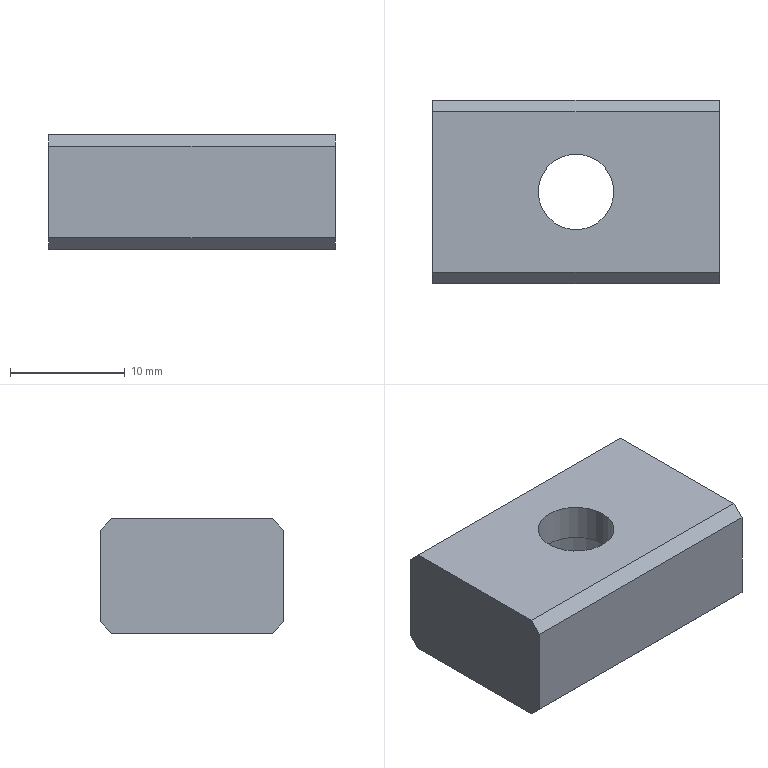Component | NX | LOCATING_KEY | 1 solid | 13 faces | box 25 x 16 x 10 mm | volume 3194 mm3 | plane 11 | cylinder 2 | commonest cylinder face diameters 6.6 x1 11 x1
STEP:
#1=CARTESIAN_POINT('',(0.,0.,0.));
#2=DIRECTION('',(0.,0.,1.));
#3=DIRECTION('',(1.,0.,0.));
#4=AXIS2_PLACEMENT_3D('',#1,#2,#3);
#5=CARTESIAN_POINT('',(225.,7.,-35.));
#6=VERTEX_POINT('',#5);
#7=CARTESIAN_POINT('',(225.,-7.,-35.));
#8=VERTEX_POINT('',#7);
#9=CARTESIAN_POINT('',(225.,8.,-35.));
#10=DIRECTION('',(0.,-1.,0.));
#11=VECTOR('',#10,1.);
#12=LINE('',#9,#11);
#13=CARTESIAN_POINT('',(225.,8.,-35.));
#14=DIRECTION('',(1.,0.,0.));
#15=DIRECTION('',(0.,0.,-1.));
#16=AXIS2_PLACEMENT_3D('',#13,#14,#15);
#17=PLANE('',#16);
#18=CARTESIAN_POINT('',(0.,0.));
#19=DIRECTION('',(0.,-1.));
#20=VECTOR('',#19,1.);
#21=LINE('',#18,#20);
#22=(GEOMETRIC_REPRESENTATION_CONTEXT(2)PARAMETRIC_REPRESENTATION_CONTEXT()REPRESENTATION_CONTEXT('',''));
#23=DEFINITIONAL_REPRESENTATION('',(#21),#22);
#24=PCURVE('',#17,#23);
#25=CARTESIAN_POINT('',(237.5,-0.,-35.));
#26=DIRECTION('',(0.,0.,1.));
#27=DIRECTION('',(1.,0.,0.));
#28=AXIS2_PLACEMENT_3D('',#25,#26,#27);
#29=PLANE('',#28);
#30=CARTESIAN_POINT('',(-12.5,8.));
#31=DIRECTION('',(0.,-1.));
#32=VECTOR('',#31,1.);
#33=LINE('',#30,#32);
#34=(GEOMETRIC_REPRESENTATION_CONTEXT(2)PARAMETRIC_REPRESENTATION_CONTEXT()REPRESENTATION_CONTEXT('',''));
#35=DEFINITIONAL_REPRESENTATION('',(#33),#34);
#36=PCURVE('',#29,#35);
#37=SURFACE_CURVE('',#12,(#24,#36),.PCURVE_S1.);
#38=EDGE_CURVE('',#6,#8,#37,.T.);
#39=ORIENTED_EDGE('',*,*,#38,.F.);
#40=CARTESIAN_POINT('',(225.,8.,-36.));
#41=VERTEX_POINT('',#40);
#42=CARTESIAN_POINT('',(225.,7.,-35.));
#43=DIRECTION('',(0.,0.7071,-0.7071));
#44=VECTOR('',#43,1.);
#45=LINE('',#42,#44);
#46=CARTESIAN_POINT('',(0.,-1.));
#47=DIRECTION('',(0.7071,0.7071));
#48=VECTOR('',#47,1.);
#49=LINE('',#46,#48);
#50=(GEOMETRIC_REPRESENTATION_CONTEXT(2)PARAMETRIC_REPRESENTATION_CONTEXT()REPRESENTATION_CONTEXT('',''));
#51=DEFINITIONAL_REPRESENTATION('',(#49),#50);
#52=PCURVE('',#17,#51);
#53=CARTESIAN_POINT('',(237.5,7.,-35.));
#54=DIRECTION('',(0.,0.7071,0.7071));
#55=DIRECTION('',(1.,0.,0.));
#56=AXIS2_PLACEMENT_3D('',#53,#54,#55);
#57=PLANE('',#56);
#58=CARTESIAN_POINT('',(-12.5,0.));
#59=DIRECTION('',(0.,1.));
#60=VECTOR('',#59,1.);
#61=LINE('',#58,#60);
#62=(GEOMETRIC_REPRESENTATION_CONTEXT(2)PARAMETRIC_REPRESENTATION_CONTEXT()REPRESENTATION_CONTEXT('',''));
#63=DEFINITIONAL_REPRESENTATION('',(#61),#62);
#64=PCURVE('',#57,#63);
#65=SURFACE_CURVE('',#45,(#52,#64),.PCURVE_S1.);
#66=EDGE_CURVE('',#6,#41,#65,.T.);
#67=ORIENTED_EDGE('',*,*,#66,.T.);
#68=CARTESIAN_POINT('',(225.,8.,-44.));
#69=VERTEX_POINT('',#68);
#70=CARTESIAN_POINT('',(225.,8.,-35.));
#71=DIRECTION('',(0.,0.,-1.));
#72=VECTOR('',#71,1.);
#73=LINE('',#70,#72);
#74=CARTESIAN_POINT('',(0.,0.));
#75=DIRECTION('',(1.,0.));
#76=VECTOR('',#75,1.);
#77=LINE('',#74,#76);
#78=(GEOMETRIC_REPRESENTATION_CONTEXT(2)PARAMETRIC_REPRESENTATION_CONTEXT()REPRESENTATION_CONTEXT('',''));
#79=DEFINITIONAL_REPRESENTATION('',(#77),#78);
#80=PCURVE('',#17,#79);
#81=CARTESIAN_POINT('',(250.,8.,-35.));
#82=DIRECTION('',(0.,-1.,0.));
#83=DIRECTION('',(0.,0.,-1.));
#84=AXIS2_PLACEMENT_3D('',#81,#82,#83);
#85=PLANE('',#84);
#86=CARTESIAN_POINT('',(0.,-25.));
#87=DIRECTION('',(1.,0.));
#88=VECTOR('',#87,1.);
#89=LINE('',#86,#88);
#90=(GEOMETRIC_REPRESENTATION_CONTEXT(2)PARAMETRIC_REPRESENTATION_CONTEXT()REPRESENTATION_CONTEXT('',''));
#91=DEFINITIONAL_REPRESENTATION('',(#89),#90);
#92=PCURVE('',#85,#91);
#93=SURFACE_CURVE('',#73,(#80,#92),.PCURVE_S1.);
#94=EDGE_CURVE('',#41,#69,#93,.T.);
#95=ORIENTED_EDGE('',*,*,#94,.T.);
#96=CARTESIAN_POINT('',(225.,7.,-45.));
#97=VERTEX_POINT('',#96);
#98=CARTESIAN_POINT('',(225.,8.,-44.));
#99=DIRECTION('',(0.,-0.7071,-0.7071));
#100=VECTOR('',#99,1.);
#101=LINE('',#98,#100);
#102=CARTESIAN_POINT('',(9.,0.));
#103=DIRECTION('',(0.7071,-0.7071));
#104=VECTOR('',#103,1.);
#105=LINE('',#102,#104);
#106=(GEOMETRIC_REPRESENTATION_CONTEXT(2)PARAMETRIC_REPRESENTATION_CONTEXT()REPRESENTATION_CONTEXT('',''));
#107=DEFINITIONAL_REPRESENTATION('',(#105),#106);
#108=PCURVE('',#17,#107);
#109=CARTESIAN_POINT('',(250.,8.,-44.));
#110=DIRECTION('',(0.,-0.7071,0.7071));
#111=DIRECTION('',(-1.,0.,0.));
#112=AXIS2_PLACEMENT_3D('',#109,#110,#111);
#113=PLANE('',#112);
#114=CARTESIAN_POINT('',(25.,0.));
#115=DIRECTION('',(0.,1.));
#116=VECTOR('',#115,1.);
#117=LINE('',#114,#116);
#118=(GEOMETRIC_REPRESENTATION_CONTEXT(2)PARAMETRIC_REPRESENTATION_CONTEXT()REPRESENTATION_CONTEXT('',''));
#119=DEFINITIONAL_REPRESENTATION('',(#117),#118);
#120=PCURVE('',#113,#119);
#121=SURFACE_CURVE('',#101,(#108,#120),.PCURVE_S1.);
#122=EDGE_CURVE('',#69,#97,#121,.T.);
#123=ORIENTED_EDGE('',*,*,#122,.T.);
#124=CARTESIAN_POINT('',(225.,-7.,-45.));
#125=VERTEX_POINT('',#124);
#126=CARTESIAN_POINT('',(225.,8.,-45.));
#127=DIRECTION('',(0.,-1.,0.));
#128=VECTOR('',#127,1.);
#129=LINE('',#126,#128);
#130=CARTESIAN_POINT('',(10.,0.));
#131=DIRECTION('',(0.,-1.));
#132=VECTOR('',#131,1.);
#133=LINE('',#130,#132);
#134=(GEOMETRIC_REPRESENTATION_CONTEXT(2)PARAMETRIC_REPRESENTATION_CONTEXT()REPRESENTATION_CONTEXT('',''));
#135=DEFINITIONAL_REPRESENTATION('',(#133),#134);
#136=PCURVE('',#17,#135);
#137=CARTESIAN_POINT('',(237.5,-0.,-45.));
#138=DIRECTION('',(0.,0.,1.));
#139=DIRECTION('',(1.,0.,0.));
#140=AXIS2_PLACEMENT_3D('',#137,#138,#139);
#141=PLANE('',#140);
#142=CARTESIAN_POINT('',(-12.5,8.));
#143=DIRECTION('',(0.,-1.));
#144=VECTOR('',#143,1.);
#145=LINE('',#142,#144);
#146=(GEOMETRIC_REPRESENTATION_CONTEXT(2)PARAMETRIC_REPRESENTATION_CONTEXT()REPRESENTATION_CONTEXT('',''));
#147=DEFINITIONAL_REPRESENTATION('',(#145),#146);
#148=PCURVE('',#141,#147);
#149=SURFACE_CURVE('',#129,(#136,#148),.PCURVE_S1.);
#150=EDGE_CURVE('',#97,#125,#149,.T.);
#151=ORIENTED_EDGE('',*,*,#150,.T.);
#152=CARTESIAN_POINT('',(225.,-8.,-44.));
#153=VERTEX_POINT('',#152);
#154=CARTESIAN_POINT('',(225.,-8.,-44.));
#155=DIRECTION('',(0.,-0.7071,0.7071));
#156=VECTOR('',#155,1.);
#157=LINE('',#154,#156);
#158=CARTESIAN_POINT('',(9.,-16.));
#159=DIRECTION('',(-0.7071,-0.7071));
#160=VECTOR('',#159,1.);
#161=LINE('',#158,#160);
#162=(GEOMETRIC_REPRESENTATION_CONTEXT(2)PARAMETRIC_REPRESENTATION_CONTEXT()REPRESENTATION_CONTEXT('',''));
#163=DEFINITIONAL_REPRESENTATION('',(#161),#162);
#164=PCURVE('',#17,#163);
#165=CARTESIAN_POINT('',(225.,-8.,-44.));
#166=DIRECTION('',(0.,0.7071,0.7071));
#167=DIRECTION('',(1.,0.,0.));
#168=AXIS2_PLACEMENT_3D('',#165,#166,#167);
#169=PLANE('',#168);
#170=CARTESIAN_POINT('',(0.,0.));
#171=DIRECTION('',(0.,-1.));
#172=VECTOR('',#171,1.);
#173=LINE('',#170,#172);
#174=(GEOMETRIC_REPRESENTATION_CONTEXT(2)PARAMETRIC_REPRESENTATION_CONTEXT()REPRESENTATION_CONTEXT('',''));
#175=DEFINITIONAL_REPRESENTATION('',(#173),#174);
#176=PCURVE('',#169,#175);
#177=SURFACE_CURVE('',#157,(#164,#176),.PCURVE_S1.);
#178=EDGE_CURVE('',#125,#153,#177,.T.);
#179=ORIENTED_EDGE('',*,*,#178,.T.);
#180=CARTESIAN_POINT('',(225.,-8.,-36.));
#181=VERTEX_POINT('',#180);
#182=CARTESIAN_POINT('',(225.,-8.,-35.));
#183=DIRECTION('',(0.,0.,-1.));
#184=VECTOR('',#183,1.);
#185=LINE('',#182,#184);
#186=CARTESIAN_POINT('',(0.,-16.));
#187=DIRECTION('',(1.,0.));
#188=VECTOR('',#187,1.);
#189=LINE('',#186,#188);
#190=(GEOMETRIC_REPRESENTATION_CONTEXT(2)PARAMETRIC_REPRESENTATION_CONTEXT()REPRESENTATION_CONTEXT('',''));
#191=DEFINITIONAL_REPRESENTATION('',(#189),#190);
#192=PCURVE('',#17,#191);
#193=CARTESIAN_POINT('',(225.,-8.,-35.));
#194=DIRECTION('',(0.,1.,0.));
#195=DIRECTION('',(0.,0.,1.));
#196=AXIS2_PLACEMENT_3D('',#193,#194,#195);
#197=PLANE('',#196);
#198=CARTESIAN_POINT('',(0.,0.));
#199=DIRECTION('',(-1.,0.));
#200=VECTOR('',#199,1.);
#201=LINE('',#198,#200);
#202=(GEOMETRIC_REPRESENTATION_CONTEXT(2)PARAMETRIC_REPRESENTATION_CONTEXT()REPRESENTATION_CONTEXT('',''));
#203=DEFINITIONAL_REPRESENTATION('',(#201),#202);
#204=PCURVE('',#197,#203);
#205=SURFACE_CURVE('',#185,(#192,#204),.PCURVE_S1.);
#206=EDGE_CURVE('',#181,#153,#205,.T.);
#207=ORIENTED_EDGE('',*,*,#206,.F.);
#208=CARTESIAN_POINT('',(225.,-7.,-35.));
#209=DIRECTION('',(0.,0.7071,0.7071));
#210=VECTOR('',#209,1.);
#211=LINE('',#208,#210);
#212=CARTESIAN_POINT('',(0.,-15.));
#213=DIRECTION('',(-0.7071,0.7071));
#214=VECTOR('',#213,1.);
#215=LINE('',#212,#214);
#216=(GEOMETRIC_REPRESENTATION_CONTEXT(2)PARAMETRIC_REPRESENTATION_CONTEXT()REPRESENTATION_CONTEXT('',''));
#217=DEFINITIONAL_REPRESENTATION('',(#215),#216);
#218=PCURVE('',#17,#217);
#219=CARTESIAN_POINT('',(237.5,-7.,-35.));
#220=DIRECTION('',(0.,-0.7071,0.7071));
#221=DIRECTION('',(-1.,0.,0.));
#222=AXIS2_PLACEMENT_3D('',#219,#220,#221);
#223=PLANE('',#222);
#224=CARTESIAN_POINT('',(12.5,0.));
#225=DIRECTION('',(0.,-1.));
#226=VECTOR('',#225,1.);
#227=LINE('',#224,#226);
#228=(GEOMETRIC_REPRESENTATION_CONTEXT(2)PARAMETRIC_REPRESENTATION_CONTEXT()REPRESENTATION_CONTEXT('',''));
#229=DEFINITIONAL_REPRESENTATION('',(#227),#228);
#230=PCURVE('',#223,#229);
#231=SURFACE_CURVE('',#211,(#218,#230),.PCURVE_S1.);
#232=EDGE_CURVE('',#181,#8,#231,.T.);
#233=ORIENTED_EDGE('',*,*,#232,.T.);
#234=EDGE_LOOP('',(#39,#67,#95,#123,#151,#179,#207,#233));
#235=FACE_BOUND('',#234,.T.);
#236=ADVANCED_FACE('',(#235),#17,.F.);
#237=ORIENTED_EDGE('',*,*,#206,.T.);
#238=CARTESIAN_POINT('',(250.,-8.,-44.));
#239=VERTEX_POINT('',#238);
#240=CARTESIAN_POINT('',(225.,-8.,-44.));
#241=DIRECTION('',(1.,0.,0.));
#242=VECTOR('',#241,1.);
#243=LINE('',#240,#242);
#244=CARTESIAN_POINT('',(-9.,0.));
#245=DIRECTION('',(0.,1.));
#246=VECTOR('',#245,1.);
#247=LINE('',#244,#246);
#248=(GEOMETRIC_REPRESENTATION_CONTEXT(2)PARAMETRIC_REPRESENTATION_CONTEXT()REPRESENTATION_CONTEXT('',''));
#249=DEFINITIONAL_REPRESENTATION('',(#247),#248);
#250=PCURVE('',#197,#249);
#251=CARTESIAN_POINT('',(0.,0.));
#252=DIRECTION('',(1.,0.));
#253=VECTOR('',#252,1.);
#254=LINE('',#251,#253);
#255=(GEOMETRIC_REPRESENTATION_CONTEXT(2)PARAMETRIC_REPRESENTATION_CONTEXT()REPRESENTATION_CONTEXT('',''));
#256=DEFINITIONAL_REPRESENTATION('',(#254),#255);
#257=PCURVE('',#169,#256);
#258=SURFACE_CURVE('',#243,(#250,#257),.PCURVE_S1.);
#259=EDGE_CURVE('',#153,#239,#258,.T.);
#260=ORIENTED_EDGE('',*,*,#259,.T.);
#261=CARTESIAN_POINT('',(250.,-8.,-36.));
#262=VERTEX_POINT('',#261);
#263=CARTESIAN_POINT('',(250.,-8.,-35.));
#264=DIRECTION('',(0.,0.,-1.));
#265=VECTOR('',#264,1.);
#266=LINE('',#263,#265);
#267=CARTESIAN_POINT('',(0.,25.));
#268=DIRECTION('',(-1.,0.));
#269=VECTOR('',#268,1.);
#270=LINE('',#267,#269);
#271=(GEOMETRIC_REPRESENTATION_CONTEXT(2)PARAMETRIC_REPRESENTATION_CONTEXT()REPRESENTATION_CONTEXT('',''));
#272=DEFINITIONAL_REPRESENTATION('',(#270),#271);
#273=PCURVE('',#197,#272);
#274=CARTESIAN_POINT('',(250.,-8.,-35.));
#275=DIRECTION('',(-1.,0.,0.));
#276=DIRECTION('',(0.,0.,1.));
#277=AXIS2_PLACEMENT_3D('',#274,#275,#276);
#278=PLANE('',#277);
#279=CARTESIAN_POINT('',(0.,0.));
#280=DIRECTION('',(-1.,0.));
#281=VECTOR('',#280,1.);
#282=LINE('',#279,#281);
#283=(GEOMETRIC_REPRESENTATION_CONTEXT(2)PARAMETRIC_REPRESENTATION_CONTEXT()REPRESENTATION_CONTEXT('',''));
#284=DEFINITIONAL_REPRESENTATION('',(#282),#283);
#285=PCURVE('',#278,#284);
#286=SURFACE_CURVE('',#266,(#273,#285),.PCURVE_S1.);
#287=EDGE_CURVE('',#262,#239,#286,.T.);
#288=ORIENTED_EDGE('',*,*,#287,.F.);
#289=CARTESIAN_POINT('',(225.,-8.,-36.));
#290=DIRECTION('',(-1.,0.,0.));
#291=VECTOR('',#290,1.);
#292=LINE('',#289,#291);
#293=CARTESIAN_POINT('',(-1.,0.));
#294=DIRECTION('',(0.,-1.));
#295=VECTOR('',#294,1.);
#296=LINE('',#293,#295);
#297=(GEOMETRIC_REPRESENTATION_CONTEXT(2)PARAMETRIC_REPRESENTATION_CONTEXT()REPRESENTATION_CONTEXT('',''));
#298=DEFINITIONAL_REPRESENTATION('',(#296),#297);
#299=PCURVE('',#197,#298);
#300=CARTESIAN_POINT('',(12.5,1.414));
#301=DIRECTION('',(1.,0.));
#302=VECTOR('',#301,1.);
#303=LINE('',#300,#302);
#304=(GEOMETRIC_REPRESENTATION_CONTEXT(2)PARAMETRIC_REPRESENTATION_CONTEXT()REPRESENTATION_CONTEXT('',''));
#305=DEFINITIONAL_REPRESENTATION('',(#303),#304);
#306=PCURVE('',#223,#305);
#307=SURFACE_CURVE('',#292,(#299,#306),.PCURVE_S1.);
#308=EDGE_CURVE('',#262,#181,#307,.T.);
#309=ORIENTED_EDGE('',*,*,#308,.T.);
#310=EDGE_LOOP('',(#237,#260,#288,#309));
#311=FACE_BOUND('',#310,.T.);
#312=ADVANCED_FACE('',(#311),#197,.F.);
#313=CARTESIAN_POINT('',(250.,8.,-36.));
#314=VERTEX_POINT('',#313);
#315=CARTESIAN_POINT('',(250.,8.,-44.));
#316=VERTEX_POINT('',#315);
#317=CARTESIAN_POINT('',(250.,8.,-35.));
#318=DIRECTION('',(0.,0.,-1.));
#319=VECTOR('',#318,1.);
#320=LINE('',#317,#319);
#321=CARTESIAN_POINT('',(0.,16.));
#322=DIRECTION('',(-1.,0.));
#323=VECTOR('',#322,1.);
#324=LINE('',#321,#323);
#325=(GEOMETRIC_REPRESENTATION_CONTEXT(2)PARAMETRIC_REPRESENTATION_CONTEXT()REPRESENTATION_CONTEXT('',''));
#326=DEFINITIONAL_REPRESENTATION('',(#324),#325);
#327=PCURVE('',#278,#326);
#328=CARTESIAN_POINT('',(0.,0.));
#329=DIRECTION('',(1.,0.));
#330=VECTOR('',#329,1.);
#331=LINE('',#328,#330);
#332=(GEOMETRIC_REPRESENTATION_CONTEXT(2)PARAMETRIC_REPRESENTATION_CONTEXT()REPRESENTATION_CONTEXT('',''));
#333=DEFINITIONAL_REPRESENTATION('',(#331),#332);
#334=PCURVE('',#85,#333);
#335=SURFACE_CURVE('',#320,(#327,#334),.PCURVE_S1.);
#336=EDGE_CURVE('',#314,#316,#335,.T.);
#337=ORIENTED_EDGE('',*,*,#336,.F.);
#338=CARTESIAN_POINT('',(250.,7.,-35.));
#339=VERTEX_POINT('',#338);
#340=CARTESIAN_POINT('',(250.,7.,-35.));
#341=DIRECTION('',(0.,-0.7071,0.7071));
#342=VECTOR('',#341,1.);
#343=LINE('',#340,#342);
#344=CARTESIAN_POINT('',(0.,15.));
#345=DIRECTION('',(0.7071,-0.7071));
#346=VECTOR('',#345,1.);
#347=LINE('',#344,#346);
#348=(GEOMETRIC_REPRESENTATION_CONTEXT(2)PARAMETRIC_REPRESENTATION_CONTEXT()REPRESENTATION_CONTEXT('',''));
#349=DEFINITIONAL_REPRESENTATION('',(#347),#348);
#350=PCURVE('',#278,#349);
#351=CARTESIAN_POINT('',(12.5,0.));
#352=DIRECTION('',(0.,-1.));
#353=VECTOR('',#352,1.);
#354=LINE('',#351,#353);
#355=(GEOMETRIC_REPRESENTATION_CONTEXT(2)PARAMETRIC_REPRESENTATION_CONTEXT()REPRESENTATION_CONTEXT('',''));
#356=DEFINITIONAL_REPRESENTATION('',(#354),#355);
#357=PCURVE('',#57,#356);
#358=SURFACE_CURVE('',#343,(#350,#357),.PCURVE_S1.);
#359=EDGE_CURVE('',#314,#339,#358,.T.);
#360=ORIENTED_EDGE('',*,*,#359,.T.);
#361=CARTESIAN_POINT('',(250.,-7.,-35.));
#362=VERTEX_POINT('',#361);
#363=CARTESIAN_POINT('',(250.,-8.,-35.));
#364=DIRECTION('',(0.,1.,0.));
#365=VECTOR('',#364,1.);
#366=LINE('',#363,#365);
#367=CARTESIAN_POINT('',(0.,0.));
#368=DIRECTION('',(0.,1.));
#369=VECTOR('',#368,1.);
#370=LINE('',#367,#369);
#371=(GEOMETRIC_REPRESENTATION_CONTEXT(2)PARAMETRIC_REPRESENTATION_CONTEXT()REPRESENTATION_CONTEXT('',''));
#372=DEFINITIONAL_REPRESENTATION('',(#370),#371);
#373=PCURVE('',#278,#372);
#374=CARTESIAN_POINT('',(12.5,-8.));
#375=DIRECTION('',(0.,1.));
#376=VECTOR('',#375,1.);
#377=LINE('',#374,#376);
#378=(GEOMETRIC_REPRESENTATION_CONTEXT(2)PARAMETRIC_REPRESENTATION_CONTEXT()REPRESENTATION_CONTEXT('',''));
#379=DEFINITIONAL_REPRESENTATION('',(#377),#378);
#380=PCURVE('',#29,#379);
#381=SURFACE_CURVE('',#366,(#373,#380),.PCURVE_S1.);
#382=EDGE_CURVE('',#362,#339,#381,.T.);
#383=ORIENTED_EDGE('',*,*,#382,.F.);
#384=CARTESIAN_POINT('',(250.,-7.,-35.));
#385=DIRECTION('',(0.,-0.7071,-0.7071));
#386=VECTOR('',#385,1.);
#387=LINE('',#384,#386);
#388=CARTESIAN_POINT('',(0.,1.));
#389=DIRECTION('',(-0.7071,-0.7071));
#390=VECTOR('',#389,1.);
#391=LINE('',#388,#390);
#392=(GEOMETRIC_REPRESENTATION_CONTEXT(2)PARAMETRIC_REPRESENTATION_CONTEXT()REPRESENTATION_CONTEXT('',''));
#393=DEFINITIONAL_REPRESENTATION('',(#391),#392);
#394=PCURVE('',#278,#393);
#395=CARTESIAN_POINT('',(-12.5,0.));
#396=DIRECTION('',(0.,1.));
#397=VECTOR('',#396,1.);
#398=LINE('',#395,#397);
#399=(GEOMETRIC_REPRESENTATION_CONTEXT(2)PARAMETRIC_REPRESENTATION_CONTEXT()REPRESENTATION_CONTEXT('',''));
#400=DEFINITIONAL_REPRESENTATION('',(#398),#399);
#401=PCURVE('',#223,#400);
#402=SURFACE_CURVE('',#387,(#394,#401),.PCURVE_S1.);
#403=EDGE_CURVE('',#362,#262,#402,.T.);
#404=ORIENTED_EDGE('',*,*,#403,.T.);
#405=ORIENTED_EDGE('',*,*,#287,.T.);
#406=CARTESIAN_POINT('',(250.,-7.,-45.));
#407=VERTEX_POINT('',#406);
#408=CARTESIAN_POINT('',(250.,-8.,-44.));
#409=DIRECTION('',(0.,0.7071,-0.7071));
#410=VECTOR('',#409,1.);
#411=LINE('',#408,#410);
#412=CARTESIAN_POINT('',(-9.,0.));
#413=DIRECTION('',(-0.7071,0.7071));
#414=VECTOR('',#413,1.);
#415=LINE('',#412,#414);
#416=(GEOMETRIC_REPRESENTATION_CONTEXT(2)PARAMETRIC_REPRESENTATION_CONTEXT()REPRESENTATION_CONTEXT('',''));
#417=DEFINITIONAL_REPRESENTATION('',(#415),#416);
#418=PCURVE('',#278,#417);
#419=CARTESIAN_POINT('',(25.,0.));
#420=DIRECTION('',(0.,1.));
#421=VECTOR('',#420,1.);
#422=LINE('',#419,#421);
#423=(GEOMETRIC_REPRESENTATION_CONTEXT(2)PARAMETRIC_REPRESENTATION_CONTEXT()REPRESENTATION_CONTEXT('',''));
#424=DEFINITIONAL_REPRESENTATION('',(#422),#423);
#425=PCURVE('',#169,#424);
#426=SURFACE_CURVE('',#411,(#418,#425),.PCURVE_S1.);
#427=EDGE_CURVE('',#239,#407,#426,.T.);
#428=ORIENTED_EDGE('',*,*,#427,.T.);
#429=CARTESIAN_POINT('',(250.,7.,-45.));
#430=VERTEX_POINT('',#429);
#431=CARTESIAN_POINT('',(250.,-8.,-45.));
#432=DIRECTION('',(0.,1.,0.));
#433=VECTOR('',#432,1.);
#434=LINE('',#431,#433);
#435=CARTESIAN_POINT('',(-10.,0.));
#436=DIRECTION('',(0.,1.));
#437=VECTOR('',#436,1.);
#438=LINE('',#435,#437);
#439=(GEOMETRIC_REPRESENTATION_CONTEXT(2)PARAMETRIC_REPRESENTATION_CONTEXT()REPRESENTATION_CONTEXT('',''));
#440=DEFINITIONAL_REPRESENTATION('',(#438),#439);
#441=PCURVE('',#278,#440);
#442=CARTESIAN_POINT('',(12.5,-8.));
#443=DIRECTION('',(0.,1.));
#444=VECTOR('',#443,1.);
#445=LINE('',#442,#444);
#446=(GEOMETRIC_REPRESENTATION_CONTEXT(2)PARAMETRIC_REPRESENTATION_CONTEXT()REPRESENTATION_CONTEXT('',''));
#447=DEFINITIONAL_REPRESENTATION('',(#445),#446);
#448=PCURVE('',#141,#447);
#449=SURFACE_CURVE('',#434,(#441,#448),.PCURVE_S1.);
#450=EDGE_CURVE('',#407,#430,#449,.T.);
#451=ORIENTED_EDGE('',*,*,#450,.T.);
#452=CARTESIAN_POINT('',(250.,8.,-44.));
#453=DIRECTION('',(0.,0.7071,0.7071));
#454=VECTOR('',#453,1.);
#455=LINE('',#452,#454);
#456=CARTESIAN_POINT('',(-9.,16.));
#457=DIRECTION('',(0.7071,0.7071));
#458=VECTOR('',#457,1.);
#459=LINE('',#456,#458);
#460=(GEOMETRIC_REPRESENTATION_CONTEXT(2)PARAMETRIC_REPRESENTATION_CONTEXT()REPRESENTATION_CONTEXT('',''));
#461=DEFINITIONAL_REPRESENTATION('',(#459),#460);
#462=PCURVE('',#278,#461);
#463=CARTESIAN_POINT('',(0.,0.));
#464=DIRECTION('',(0.,-1.));
#465=VECTOR('',#464,1.);
#466=LINE('',#463,#465);
#467=(GEOMETRIC_REPRESENTATION_CONTEXT(2)PARAMETRIC_REPRESENTATION_CONTEXT()REPRESENTATION_CONTEXT('',''));
#468=DEFINITIONAL_REPRESENTATION('',(#466),#467);
#469=PCURVE('',#113,#468);
#470=SURFACE_CURVE('',#455,(#462,#469),.PCURVE_S1.);
#471=EDGE_CURVE('',#430,#316,#470,.T.);
#472=ORIENTED_EDGE('',*,*,#471,.T.);
#473=EDGE_LOOP('',(#337,#360,#383,#404,#405,#428,#451,#472));
#474=FACE_BOUND('',#473,.T.);
#475=ADVANCED_FACE('',(#474),#278,.F.);
#476=ORIENTED_EDGE('',*,*,#94,.F.);
#477=CARTESIAN_POINT('',(250.,8.,-36.));
#478=DIRECTION('',(1.,0.,0.));
#479=VECTOR('',#478,1.);
#480=LINE('',#477,#479);
#481=CARTESIAN_POINT('',(1.,0.));
#482=DIRECTION('',(0.,1.));
#483=VECTOR('',#482,1.);
#484=LINE('',#481,#483);
#485=(GEOMETRIC_REPRESENTATION_CONTEXT(2)PARAMETRIC_REPRESENTATION_CONTEXT()REPRESENTATION_CONTEXT('',''));
#486=DEFINITIONAL_REPRESENTATION('',(#484),#485);
#487=PCURVE('',#85,#486);
#488=CARTESIAN_POINT('',(12.5,1.414));
#489=DIRECTION('',(1.,0.));
#490=VECTOR('',#489,1.);
#491=LINE('',#488,#490);
#492=(GEOMETRIC_REPRESENTATION_CONTEXT(2)PARAMETRIC_REPRESENTATION_CONTEXT()REPRESENTATION_CONTEXT('',''));
#493=DEFINITIONAL_REPRESENTATION('',(#491),#492);
#494=PCURVE('',#57,#493);
#495=SURFACE_CURVE('',#480,(#487,#494),.PCURVE_S1.);
#496=EDGE_CURVE('',#41,#314,#495,.T.);
#497=ORIENTED_EDGE('',*,*,#496,.T.);
#498=ORIENTED_EDGE('',*,*,#336,.T.);
#499=CARTESIAN_POINT('',(250.,8.,-44.));
#500=DIRECTION('',(-1.,0.,0.));
#501=VECTOR('',#500,1.);
#502=LINE('',#499,#501);
#503=CARTESIAN_POINT('',(9.,0.));
#504=DIRECTION('',(0.,-1.));
#505=VECTOR('',#504,1.);
#506=LINE('',#503,#505);
#507=(GEOMETRIC_REPRESENTATION_CONTEXT(2)PARAMETRIC_REPRESENTATION_CONTEXT()REPRESENTATION_CONTEXT('',''));
#508=DEFINITIONAL_REPRESENTATION('',(#506),#507);
#509=PCURVE('',#85,#508);
#510=CARTESIAN_POINT('',(0.,0.));
#511=DIRECTION('',(1.,0.));
#512=VECTOR('',#511,1.);
#513=LINE('',#510,#512);
#514=(GEOMETRIC_REPRESENTATION_CONTEXT(2)PARAMETRIC_REPRESENTATION_CONTEXT()REPRESENTATION_CONTEXT('',''));
#515=DEFINITIONAL_REPRESENTATION('',(#513),#514);
#516=PCURVE('',#113,#515);
#517=SURFACE_CURVE('',#502,(#509,#516),.PCURVE_S1.);
#518=EDGE_CURVE('',#316,#69,#517,.T.);
#519=ORIENTED_EDGE('',*,*,#518,.T.);
#520=EDGE_LOOP('',(#476,#497,#498,#519));
#521=FACE_BOUND('',#520,.T.);
#522=ADVANCED_FACE('',(#521),#85,.F.);
#523=CARTESIAN_POINT('',(240.8,-0.,-35.));
#524=VERTEX_POINT('',#523);
#525=CARTESIAN_POINT('',(237.5,-0.,-35.));
#526=DIRECTION('',(0.,0.,1.));
#527=DIRECTION('',(1.,0.,0.));
#528=AXIS2_PLACEMENT_3D('',#525,#526,#527);
#529=CIRCLE('',#528,3.3);
#530=CARTESIAN_POINT('',(0.,0.));
#531=DIRECTION('',(1.,0.));
#532=AXIS2_PLACEMENT_2D('',#530,#531);
#533=CIRCLE('',#532,3.3);
#534=(GEOMETRIC_REPRESENTATION_CONTEXT(2)PARAMETRIC_REPRESENTATION_CONTEXT()REPRESENTATION_CONTEXT('',''));
#535=DEFINITIONAL_REPRESENTATION('',(#533),#534);
#536=PCURVE('',#29,#535);
#537=CARTESIAN_POINT('',(237.5,-0.,-22.773));
#538=DIRECTION('',(0.,0.,1.));
#539=DIRECTION('',(1.,0.,0.));
#540=AXIS2_PLACEMENT_3D('',#537,#538,#539);
#541=CYLINDRICAL_SURFACE('',#540,3.3);
#542=CARTESIAN_POINT('',(0.,-12.227));
#543=DIRECTION('',(1.,0.));
#544=VECTOR('',#543,1.);
#545=LINE('',#542,#544);
#546=(GEOMETRIC_REPRESENTATION_CONTEXT(2)PARAMETRIC_REPRESENTATION_CONTEXT()REPRESENTATION_CONTEXT('',''));
#547=DEFINITIONAL_REPRESENTATION('',(#545),#546);
#548=PCURVE('',#541,#547);
#549=SURFACE_CURVE('',#529,(#536,#548),.PCURVE_S1.);
#550=EDGE_CURVE('',#524,#524,#549,.T.);
#551=ORIENTED_EDGE('',*,*,#550,.F.);
#552=EDGE_LOOP('',(#551));
#553=FACE_BOUND('',#552,.T.);
#554=ORIENTED_EDGE('',*,*,#382,.T.);
#555=CARTESIAN_POINT('',(225.,7.,-35.));
#556=DIRECTION('',(-1.,0.,0.));
#557=VECTOR('',#556,1.);
#558=LINE('',#555,#557);
#559=CARTESIAN_POINT('',(-12.5,7.));
#560=DIRECTION('',(-1.,0.));
#561=VECTOR('',#560,1.);
#562=LINE('',#559,#561);
#563=(GEOMETRIC_REPRESENTATION_CONTEXT(2)PARAMETRIC_REPRESENTATION_CONTEXT()REPRESENTATION_CONTEXT('',''));
#564=DEFINITIONAL_REPRESENTATION('',(#562),#563);
#565=PCURVE('',#29,#564);
#566=CARTESIAN_POINT('',(-12.5,0.));
#567=DIRECTION('',(-1.,0.));
#568=VECTOR('',#567,1.);
#569=LINE('',#566,#568);
#570=(GEOMETRIC_REPRESENTATION_CONTEXT(2)PARAMETRIC_REPRESENTATION_CONTEXT()REPRESENTATION_CONTEXT('',''));
#571=DEFINITIONAL_REPRESENTATION('',(#569),#570);
#572=PCURVE('',#57,#571);
#573=SURFACE_CURVE('',#558,(#565,#572),.PCURVE_S1.);
#574=EDGE_CURVE('',#339,#6,#573,.T.);
#575=ORIENTED_EDGE('',*,*,#574,.T.);
#576=ORIENTED_EDGE('',*,*,#38,.T.);
#577=CARTESIAN_POINT('',(250.,-7.,-35.));
#578=DIRECTION('',(1.,0.,0.));
#579=VECTOR('',#578,1.);
#580=LINE('',#577,#579);
#581=CARTESIAN_POINT('',(12.5,-7.));
#582=DIRECTION('',(1.,0.));
#583=VECTOR('',#582,1.);
#584=LINE('',#581,#583);
#585=(GEOMETRIC_REPRESENTATION_CONTEXT(2)PARAMETRIC_REPRESENTATION_CONTEXT()REPRESENTATION_CONTEXT('',''));
#586=DEFINITIONAL_REPRESENTATION('',(#584),#585);
#587=PCURVE('',#29,#586);
#588=CARTESIAN_POINT('',(-12.5,0.));
#589=DIRECTION('',(-1.,0.));
#590=VECTOR('',#589,1.);
#591=LINE('',#588,#590);
#592=(GEOMETRIC_REPRESENTATION_CONTEXT(2)PARAMETRIC_REPRESENTATION_CONTEXT()REPRESENTATION_CONTEXT('',''));
#593=DEFINITIONAL_REPRESENTATION('',(#591),#592);
#594=PCURVE('',#223,#593);
#595=SURFACE_CURVE('',#580,(#587,#594),.PCURVE_S1.);
#596=EDGE_CURVE('',#8,#362,#595,.T.);
#597=ORIENTED_EDGE('',*,*,#596,.T.);
#598=EDGE_LOOP('',(#554,#575,#576,#597));
#599=FACE_BOUND('',#598,.T.);
#600=ADVANCED_FACE('',(#553,#599),#29,.T.);
#601=CARTESIAN_POINT('',(243.,-0.,-45.));
#602=VERTEX_POINT('',#601);
#603=CARTESIAN_POINT('',(237.5,-0.,-45.));
#604=DIRECTION('',(0.,0.,1.));
#605=DIRECTION('',(1.,0.,0.));
#606=AXIS2_PLACEMENT_3D('',#603,#604,#605);
#607=CIRCLE('',#606,5.5);
#608=CARTESIAN_POINT('',(0.,0.));
#609=DIRECTION('',(1.,0.));
#610=AXIS2_PLACEMENT_2D('',#608,#609);
#611=CIRCLE('',#610,5.5);
#612=(GEOMETRIC_REPRESENTATION_CONTEXT(2)PARAMETRIC_REPRESENTATION_CONTEXT()REPRESENTATION_CONTEXT('',''));
#613=DEFINITIONAL_REPRESENTATION('',(#611),#612);
#614=PCURVE('',#141,#613);
#615=CARTESIAN_POINT('',(237.5,-0.,-45.));
#616=DIRECTION('',(0.,0.,1.));
#617=DIRECTION('',(1.,0.,0.));
#618=AXIS2_PLACEMENT_3D('',#615,#616,#617);
#619=CYLINDRICAL_SURFACE('',#618,5.5);
#620=CARTESIAN_POINT('',(0.,0.));
#621=DIRECTION('',(1.,0.));
#622=VECTOR('',#621,1.);
#623=LINE('',#620,#622);
#624=(GEOMETRIC_REPRESENTATION_CONTEXT(2)PARAMETRIC_REPRESENTATION_CONTEXT()REPRESENTATION_CONTEXT('',''));
#625=DEFINITIONAL_REPRESENTATION('',(#623),#624);
#626=PCURVE('',#619,#625);
#627=SURFACE_CURVE('',#607,(#614,#626),.PCURVE_S1.);
#628=EDGE_CURVE('',#602,#602,#627,.T.);
#629=ORIENTED_EDGE('',*,*,#628,.T.);
#630=EDGE_LOOP('',(#629));
#631=FACE_BOUND('',#630,.T.);
#632=ORIENTED_EDGE('',*,*,#150,.F.);
#633=CARTESIAN_POINT('',(237.5,7.,-45.));
#634=DIRECTION('',(1.,0.,0.));
#635=VECTOR('',#634,1.);
#636=LINE('',#633,#635);
#637=CARTESIAN_POINT('',(0.,7.));
#638=DIRECTION('',(1.,0.));
#639=VECTOR('',#638,1.);
#640=LINE('',#637,#639);
#641=(GEOMETRIC_REPRESENTATION_CONTEXT(2)PARAMETRIC_REPRESENTATION_CONTEXT()REPRESENTATION_CONTEXT('',''));
#642=DEFINITIONAL_REPRESENTATION('',(#640),#641);
#643=PCURVE('',#141,#642);
#644=CARTESIAN_POINT('',(12.5,1.414));
#645=DIRECTION('',(-1.,0.));
#646=VECTOR('',#645,1.);
#647=LINE('',#644,#646);
#648=(GEOMETRIC_REPRESENTATION_CONTEXT(2)PARAMETRIC_REPRESENTATION_CONTEXT()REPRESENTATION_CONTEXT('',''));
#649=DEFINITIONAL_REPRESENTATION('',(#647),#648);
#650=PCURVE('',#113,#649);
#651=SURFACE_CURVE('',#636,(#643,#650),.PCURVE_S1.);
#652=EDGE_CURVE('',#97,#430,#651,.T.);
#653=ORIENTED_EDGE('',*,*,#652,.T.);
#654=ORIENTED_EDGE('',*,*,#450,.F.);
#655=CARTESIAN_POINT('',(237.5,-7.,-45.));
#656=DIRECTION('',(-1.,0.,0.));
#657=VECTOR('',#656,1.);
#658=LINE('',#655,#657);
#659=CARTESIAN_POINT('',(0.,-7.));
#660=DIRECTION('',(-1.,0.));
#661=VECTOR('',#660,1.);
#662=LINE('',#659,#661);
#663=(GEOMETRIC_REPRESENTATION_CONTEXT(2)PARAMETRIC_REPRESENTATION_CONTEXT()REPRESENTATION_CONTEXT('',''));
#664=DEFINITIONAL_REPRESENTATION('',(#662),#663);
#665=PCURVE('',#141,#664);
#666=CARTESIAN_POINT('',(12.5,1.414));
#667=DIRECTION('',(-1.,0.));
#668=VECTOR('',#667,1.);
#669=LINE('',#666,#668);
#670=(GEOMETRIC_REPRESENTATION_CONTEXT(2)PARAMETRIC_REPRESENTATION_CONTEXT()REPRESENTATION_CONTEXT('',''));
#671=DEFINITIONAL_REPRESENTATION('',(#669),#670);
#672=PCURVE('',#169,#671);
#673=SURFACE_CURVE('',#658,(#665,#672),.PCURVE_S1.);
#674=EDGE_CURVE('',#407,#125,#673,.T.);
#675=ORIENTED_EDGE('',*,*,#674,.T.);
#676=EDGE_LOOP('',(#632,#653,#654,#675));
#677=FACE_BOUND('',#676,.T.);
#678=ADVANCED_FACE('',(#631,#677),#141,.F.);
#679=ORIENTED_EDGE('',*,*,#550,.F.);
#680=CARTESIAN_POINT('',(240.8,-0.,-38.2));
#681=VERTEX_POINT('',#680);
#682=CARTESIAN_POINT('',(240.8,-0.,-38.2));
#683=CARTESIAN_POINT('',(240.8,-0.,-35.));
#684=B_SPLINE_CURVE_WITH_KNOTS('',1,(#682,#683),.UNSPECIFIED.,.F.,.F.,(2,2),(-15.427,-12.227),.PIECEWISE_BEZIER_KNOTS.);
#685=CARTESIAN_POINT('',(0.,0.));
#686=DIRECTION('',(0.,1.));
#687=VECTOR('',#686,1.);
#688=LINE('',#685,#687);
#689=(GEOMETRIC_REPRESENTATION_CONTEXT(2)PARAMETRIC_REPRESENTATION_CONTEXT()REPRESENTATION_CONTEXT('',''));
#690=DEFINITIONAL_REPRESENTATION('',(#688),#689);
#691=PCURVE('',#541,#690);
#692=CARTESIAN_POINT('',(6.283,0.));
#693=DIRECTION('',(0.,1.));
#694=VECTOR('',#693,1.);
#695=LINE('',#692,#694);
#696=(GEOMETRIC_REPRESENTATION_CONTEXT(2)PARAMETRIC_REPRESENTATION_CONTEXT()REPRESENTATION_CONTEXT('',''));
#697=DEFINITIONAL_REPRESENTATION('',(#695),#696);
#698=PCURVE('',#541,#697);
#699=SEAM_CURVE('',#684,(#691,#698),.PCURVE_S1.);
#700=EDGE_CURVE('',#681,#524,#699,.T.);
#701=ORIENTED_EDGE('',*,*,#700,.F.);
#702=CARTESIAN_POINT('',(237.5,-0.,-38.2));
#703=DIRECTION('',(0.,0.,-1.));
#704=DIRECTION('',(1.,0.,0.));
#705=AXIS2_PLACEMENT_3D('',#702,#703,#704);
#706=CIRCLE('',#705,3.3);
#707=CARTESIAN_POINT('',(6.283,-15.427));
#708=DIRECTION('',(-1.,0.));
#709=VECTOR('',#708,1.);
#710=LINE('',#707,#709);
#711=(GEOMETRIC_REPRESENTATION_CONTEXT(2)PARAMETRIC_REPRESENTATION_CONTEXT()REPRESENTATION_CONTEXT('',''));
#712=DEFINITIONAL_REPRESENTATION('',(#710),#711);
#713=PCURVE('',#541,#712);
#714=CARTESIAN_POINT('',(237.5,-0.,-38.2));
#715=DIRECTION('',(0.,0.,1.));
#716=DIRECTION('',(1.,0.,0.));
#717=AXIS2_PLACEMENT_3D('',#714,#715,#716);
#718=PLANE('',#717);
#719=CARTESIAN_POINT('',(3.3,0.));
#720=CARTESIAN_POINT('',(3.3,-5.716));
#721=CARTESIAN_POINT('',(-1.65,-2.858));
#722=CARTESIAN_POINT('',(-6.6,-0.));
#723=CARTESIAN_POINT('',(-1.65,2.858));
#724=CARTESIAN_POINT('',(3.3,5.716));
#725=CARTESIAN_POINT('',(3.3,0.));
#726=(BOUNDED_CURVE()B_SPLINE_CURVE(2,(#719,#720,#721,#722,#723,#724,#725),.UNSPECIFIED.,.T.,.F.)B_SPLINE_CURVE_WITH_KNOTS((1,2,2,2,2,1),(-2.094,0.,2.094,4.189,6.283,8.378),.UNSPECIFIED.)CURVE()GEOMETRIC_REPRESENTATION_ITEM()RATIONAL_B_SPLINE_CURVE((1.,0.5,1.,0.5,1.,0.5,1.))REPRESENTATION_ITEM(''));
#727=(GEOMETRIC_REPRESENTATION_CONTEXT(2)PARAMETRIC_REPRESENTATION_CONTEXT()REPRESENTATION_CONTEXT('',''));
#728=DEFINITIONAL_REPRESENTATION('',(#726),#727);
#729=PCURVE('',#718,#728);
#730=SURFACE_CURVE('',#706,(#713,#729),.PCURVE_S1.);
#731=EDGE_CURVE('',#681,#681,#730,.T.);
#732=ORIENTED_EDGE('',*,*,#731,.F.);
#733=ORIENTED_EDGE('',*,*,#700,.T.);
#734=EDGE_LOOP('',(#679,#701,#732,#733));
#735=FACE_BOUND('',#734,.F.);
#736=ADVANCED_FACE('',(#735),#541,.F.);
#737=ORIENTED_EDGE('',*,*,#731,.F.);
#738=EDGE_LOOP('',(#737));
#739=FACE_BOUND('',#738,.T.);
#740=CARTESIAN_POINT('',(243.,-0.,-38.2));
#741=VERTEX_POINT('',#740);
#742=CARTESIAN_POINT('',(237.5,-0.,-38.2));
#743=DIRECTION('',(0.,0.,-1.));
#744=DIRECTION('',(1.,0.,0.));
#745=AXIS2_PLACEMENT_3D('',#742,#743,#744);
#746=CIRCLE('',#745,5.5);
#747=CARTESIAN_POINT('',(5.5,0.));
#748=CARTESIAN_POINT('',(5.5,-9.526));
#749=CARTESIAN_POINT('',(-2.75,-4.763));
#750=CARTESIAN_POINT('',(-11.,-0.));
#751=CARTESIAN_POINT('',(-2.75,4.763));
#752=CARTESIAN_POINT('',(5.5,9.526));
#753=CARTESIAN_POINT('',(5.5,0.));
#754=(BOUNDED_CURVE()B_SPLINE_CURVE(2,(#747,#748,#749,#750,#751,#752,#753),.UNSPECIFIED.,.T.,.F.)B_SPLINE_CURVE_WITH_KNOTS((1,2,2,2,2,1),(-2.094,0.,2.094,4.189,6.283,8.378),.UNSPECIFIED.)CURVE()GEOMETRIC_REPRESENTATION_ITEM()RATIONAL_B_SPLINE_CURVE((1.,0.5,1.,0.5,1.,0.5,1.))REPRESENTATION_ITEM(''));
#755=(GEOMETRIC_REPRESENTATION_CONTEXT(2)PARAMETRIC_REPRESENTATION_CONTEXT()REPRESENTATION_CONTEXT('',''));
#756=DEFINITIONAL_REPRESENTATION('',(#754),#755);
#757=PCURVE('',#718,#756);
#758=CARTESIAN_POINT('',(6.283,6.8));
#759=DIRECTION('',(-1.,0.));
#760=VECTOR('',#759,1.);
#761=LINE('',#758,#760);
#762=(GEOMETRIC_REPRESENTATION_CONTEXT(2)PARAMETRIC_REPRESENTATION_CONTEXT()REPRESENTATION_CONTEXT('',''));
#763=DEFINITIONAL_REPRESENTATION('',(#761),#762);
#764=PCURVE('',#619,#763);
#765=SURFACE_CURVE('',#746,(#757,#764),.PCURVE_S1.);
#766=EDGE_CURVE('',#741,#741,#765,.T.);
#767=ORIENTED_EDGE('',*,*,#766,.T.);
#768=EDGE_LOOP('',(#767));
#769=FACE_BOUND('',#768,.T.);
#770=ADVANCED_FACE('',(#739,#769),#718,.F.);
#771=ORIENTED_EDGE('',*,*,#766,.T.);
#772=CARTESIAN_POINT('',(243.,-0.,-45.));
#773=CARTESIAN_POINT('',(243.,-0.,-38.2));
#774=B_SPLINE_CURVE_WITH_KNOTS('',1,(#772,#773),.UNSPECIFIED.,.F.,.F.,(2,2),(0.,6.8),.PIECEWISE_BEZIER_KNOTS.);
#775=CARTESIAN_POINT('',(0.,0.));
#776=DIRECTION('',(0.,1.));
#777=VECTOR('',#776,1.);
#778=LINE('',#775,#777);
#779=(GEOMETRIC_REPRESENTATION_CONTEXT(2)PARAMETRIC_REPRESENTATION_CONTEXT()REPRESENTATION_CONTEXT('',''));
#780=DEFINITIONAL_REPRESENTATION('',(#778),#779);
#781=PCURVE('',#619,#780);
#782=CARTESIAN_POINT('',(6.283,0.));
#783=DIRECTION('',(0.,1.));
#784=VECTOR('',#783,1.);
#785=LINE('',#782,#784);
#786=(GEOMETRIC_REPRESENTATION_CONTEXT(2)PARAMETRIC_REPRESENTATION_CONTEXT()REPRESENTATION_CONTEXT('',''));
#787=DEFINITIONAL_REPRESENTATION('',(#785),#786);
#788=PCURVE('',#619,#787);
#789=SEAM_CURVE('',#774,(#781,#788),.PCURVE_S1.);
#790=EDGE_CURVE('',#602,#741,#789,.T.);
#791=ORIENTED_EDGE('',*,*,#790,.F.);
#792=ORIENTED_EDGE('',*,*,#628,.T.);
#793=ORIENTED_EDGE('',*,*,#790,.T.);
#794=EDGE_LOOP('',(#771,#791,#792,#793));
#795=FACE_BOUND('',#794,.F.);
#796=ADVANCED_FACE('',(#795),#619,.F.);
#797=ORIENTED_EDGE('',*,*,#359,.F.);
#798=ORIENTED_EDGE('',*,*,#496,.F.);
#799=ORIENTED_EDGE('',*,*,#66,.F.);
#800=ORIENTED_EDGE('',*,*,#574,.F.);
#801=EDGE_LOOP('',(#797,#798,#799,#800));
#802=FACE_BOUND('',#801,.T.);
#803=ADVANCED_FACE('',(#802),#57,.T.);
#804=ORIENTED_EDGE('',*,*,#471,.F.);
#805=ORIENTED_EDGE('',*,*,#652,.F.);
#806=ORIENTED_EDGE('',*,*,#122,.F.);
#807=ORIENTED_EDGE('',*,*,#518,.F.);
#808=EDGE_LOOP('',(#804,#805,#806,#807));
#809=FACE_BOUND('',#808,.T.);
#810=ADVANCED_FACE('',(#809),#113,.F.);
#811=ORIENTED_EDGE('',*,*,#178,.F.);
#812=ORIENTED_EDGE('',*,*,#674,.F.);
#813=ORIENTED_EDGE('',*,*,#427,.F.);
#814=ORIENTED_EDGE('',*,*,#259,.F.);
#815=EDGE_LOOP('',(#811,#812,#813,#814));
#816=FACE_BOUND('',#815,.T.);
#817=ADVANCED_FACE('',(#816),#169,.F.);
#818=ORIENTED_EDGE('',*,*,#232,.F.);
#819=ORIENTED_EDGE('',*,*,#308,.F.);
#820=ORIENTED_EDGE('',*,*,#403,.F.);
#821=ORIENTED_EDGE('',*,*,#596,.F.);
#822=EDGE_LOOP('',(#818,#819,#820,#821));
#823=FACE_BOUND('',#822,.T.);
#824=ADVANCED_FACE('',(#823),#223,.T.);
#825=CLOSED_SHELL('',(#236,#312,#475,#522,#600,#678,#736,#770,#796,#803,#810,#817,#824));
#826=MANIFOLD_SOLID_BREP('',#825);
#827=(LENGTH_UNIT()NAMED_UNIT(*)SI_UNIT(.MILLI.,.METRE.));
#828=UNCERTAINTY_MEASURE_WITH_UNIT(LENGTH_MEASURE(0.000002),#827,'','');
#829=(NAMED_UNIT(*)PLANE_ANGLE_UNIT()SI_UNIT($,.RADIAN.));
#830=(NAMED_UNIT(*)SI_UNIT($,.STERADIAN.)SOLID_ANGLE_UNIT());
#831=(GEOMETRIC_REPRESENTATION_CONTEXT(3)GLOBAL_UNCERTAINTY_ASSIGNED_CONTEXT((#828))GLOBAL_UNIT_ASSIGNED_CONTEXT((#827,#829,#830))REPRESENTATION_CONTEXT('',''));
#832=ADVANCED_BREP_SHAPE_REPRESENTATION('',(#4,#826),#831);